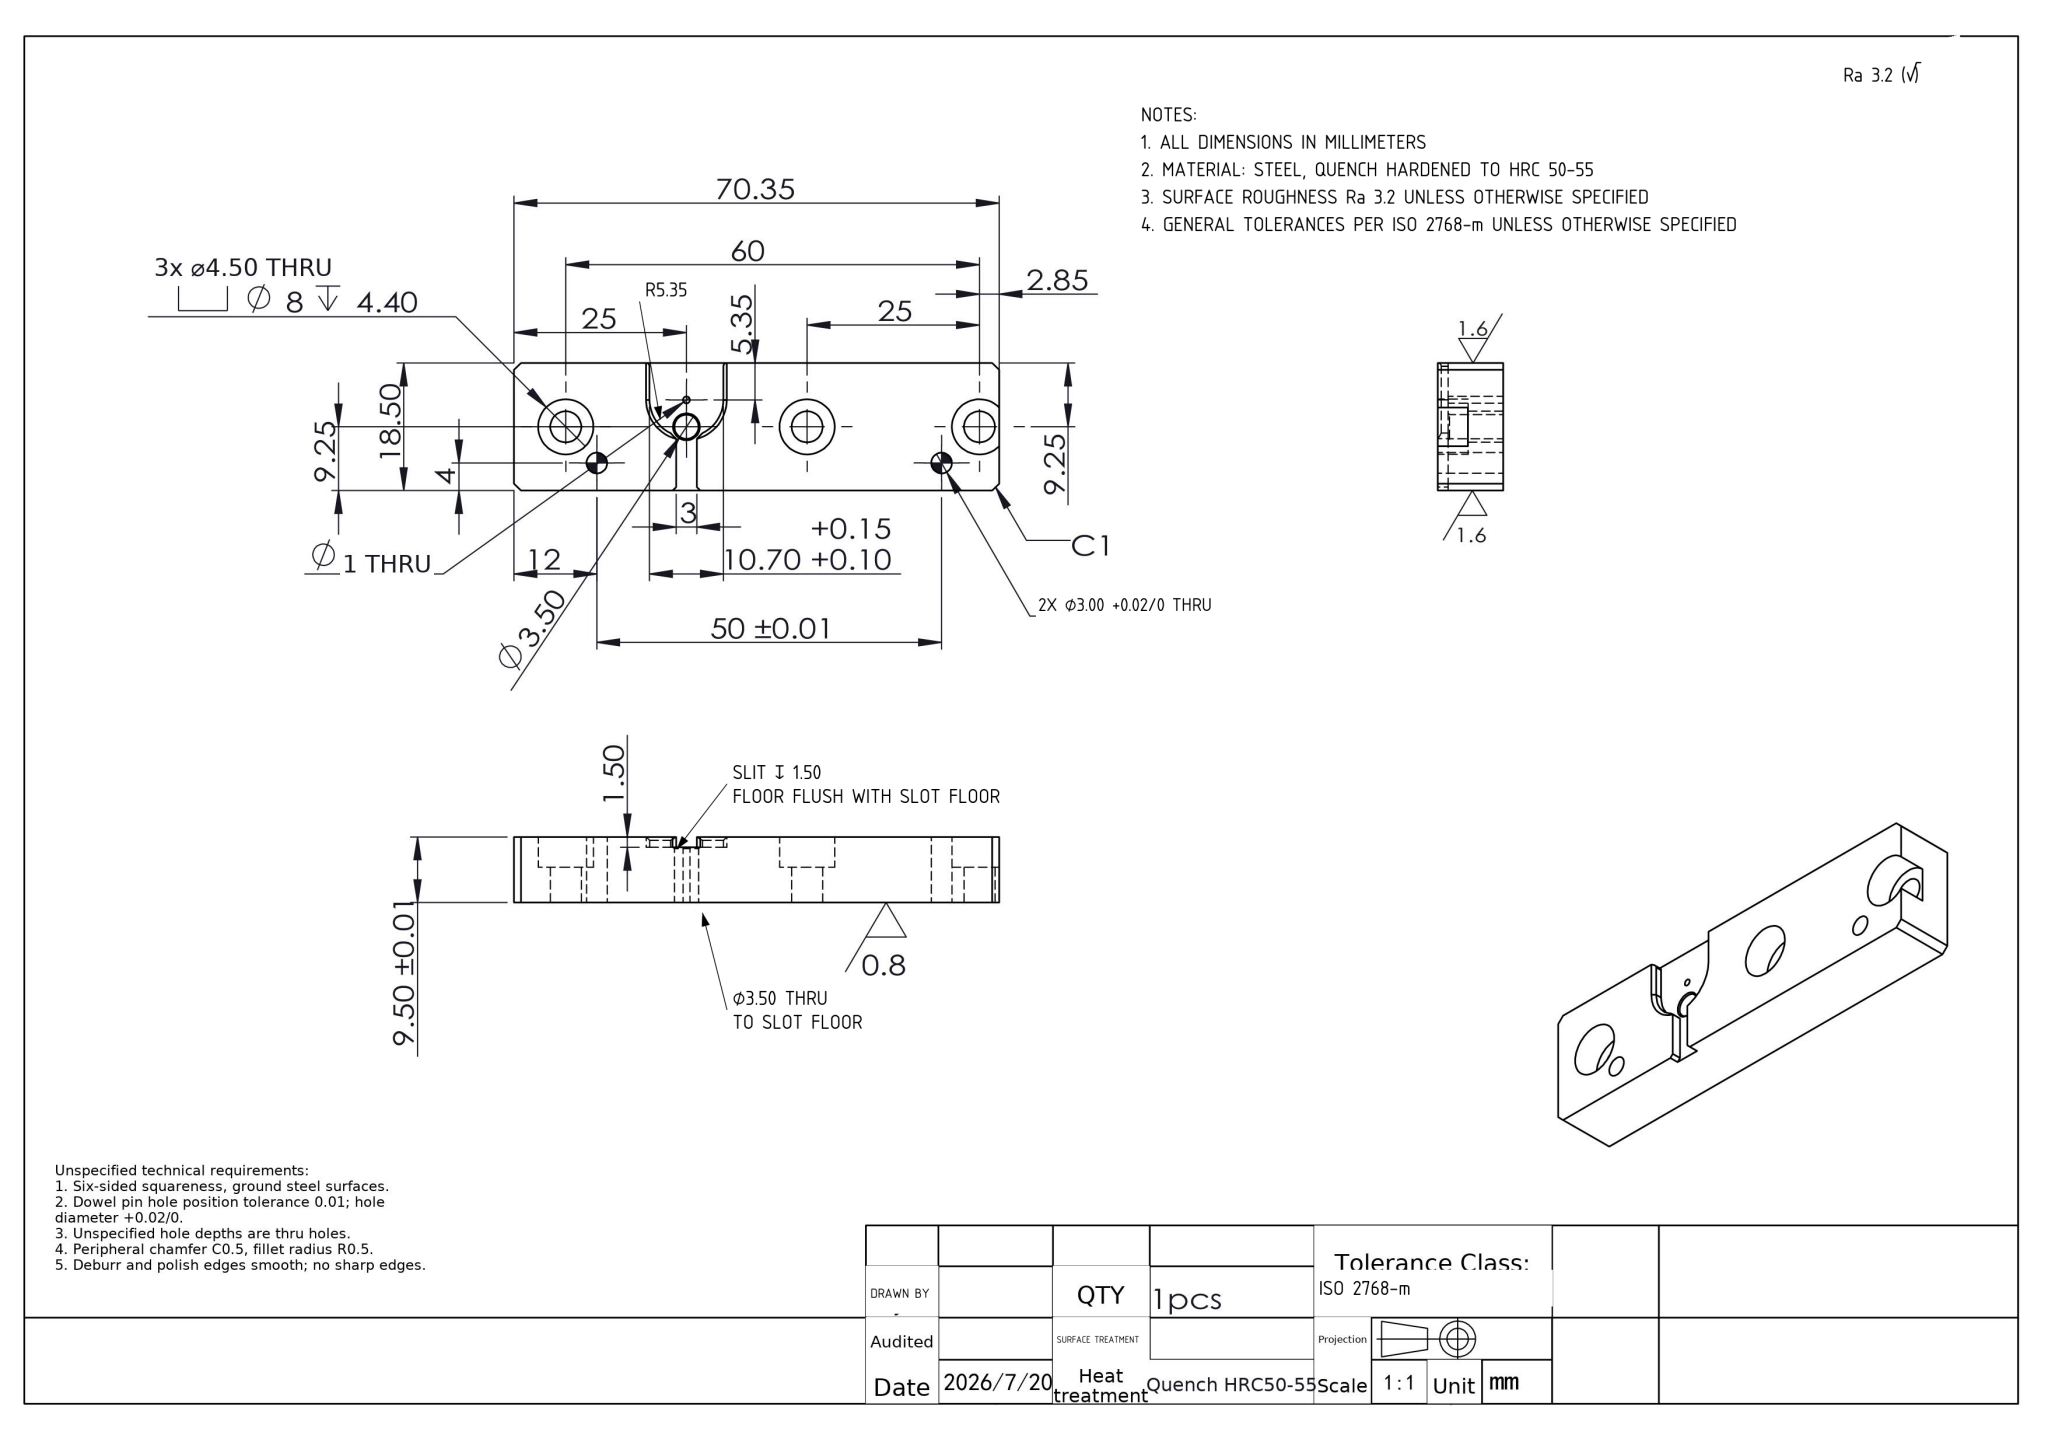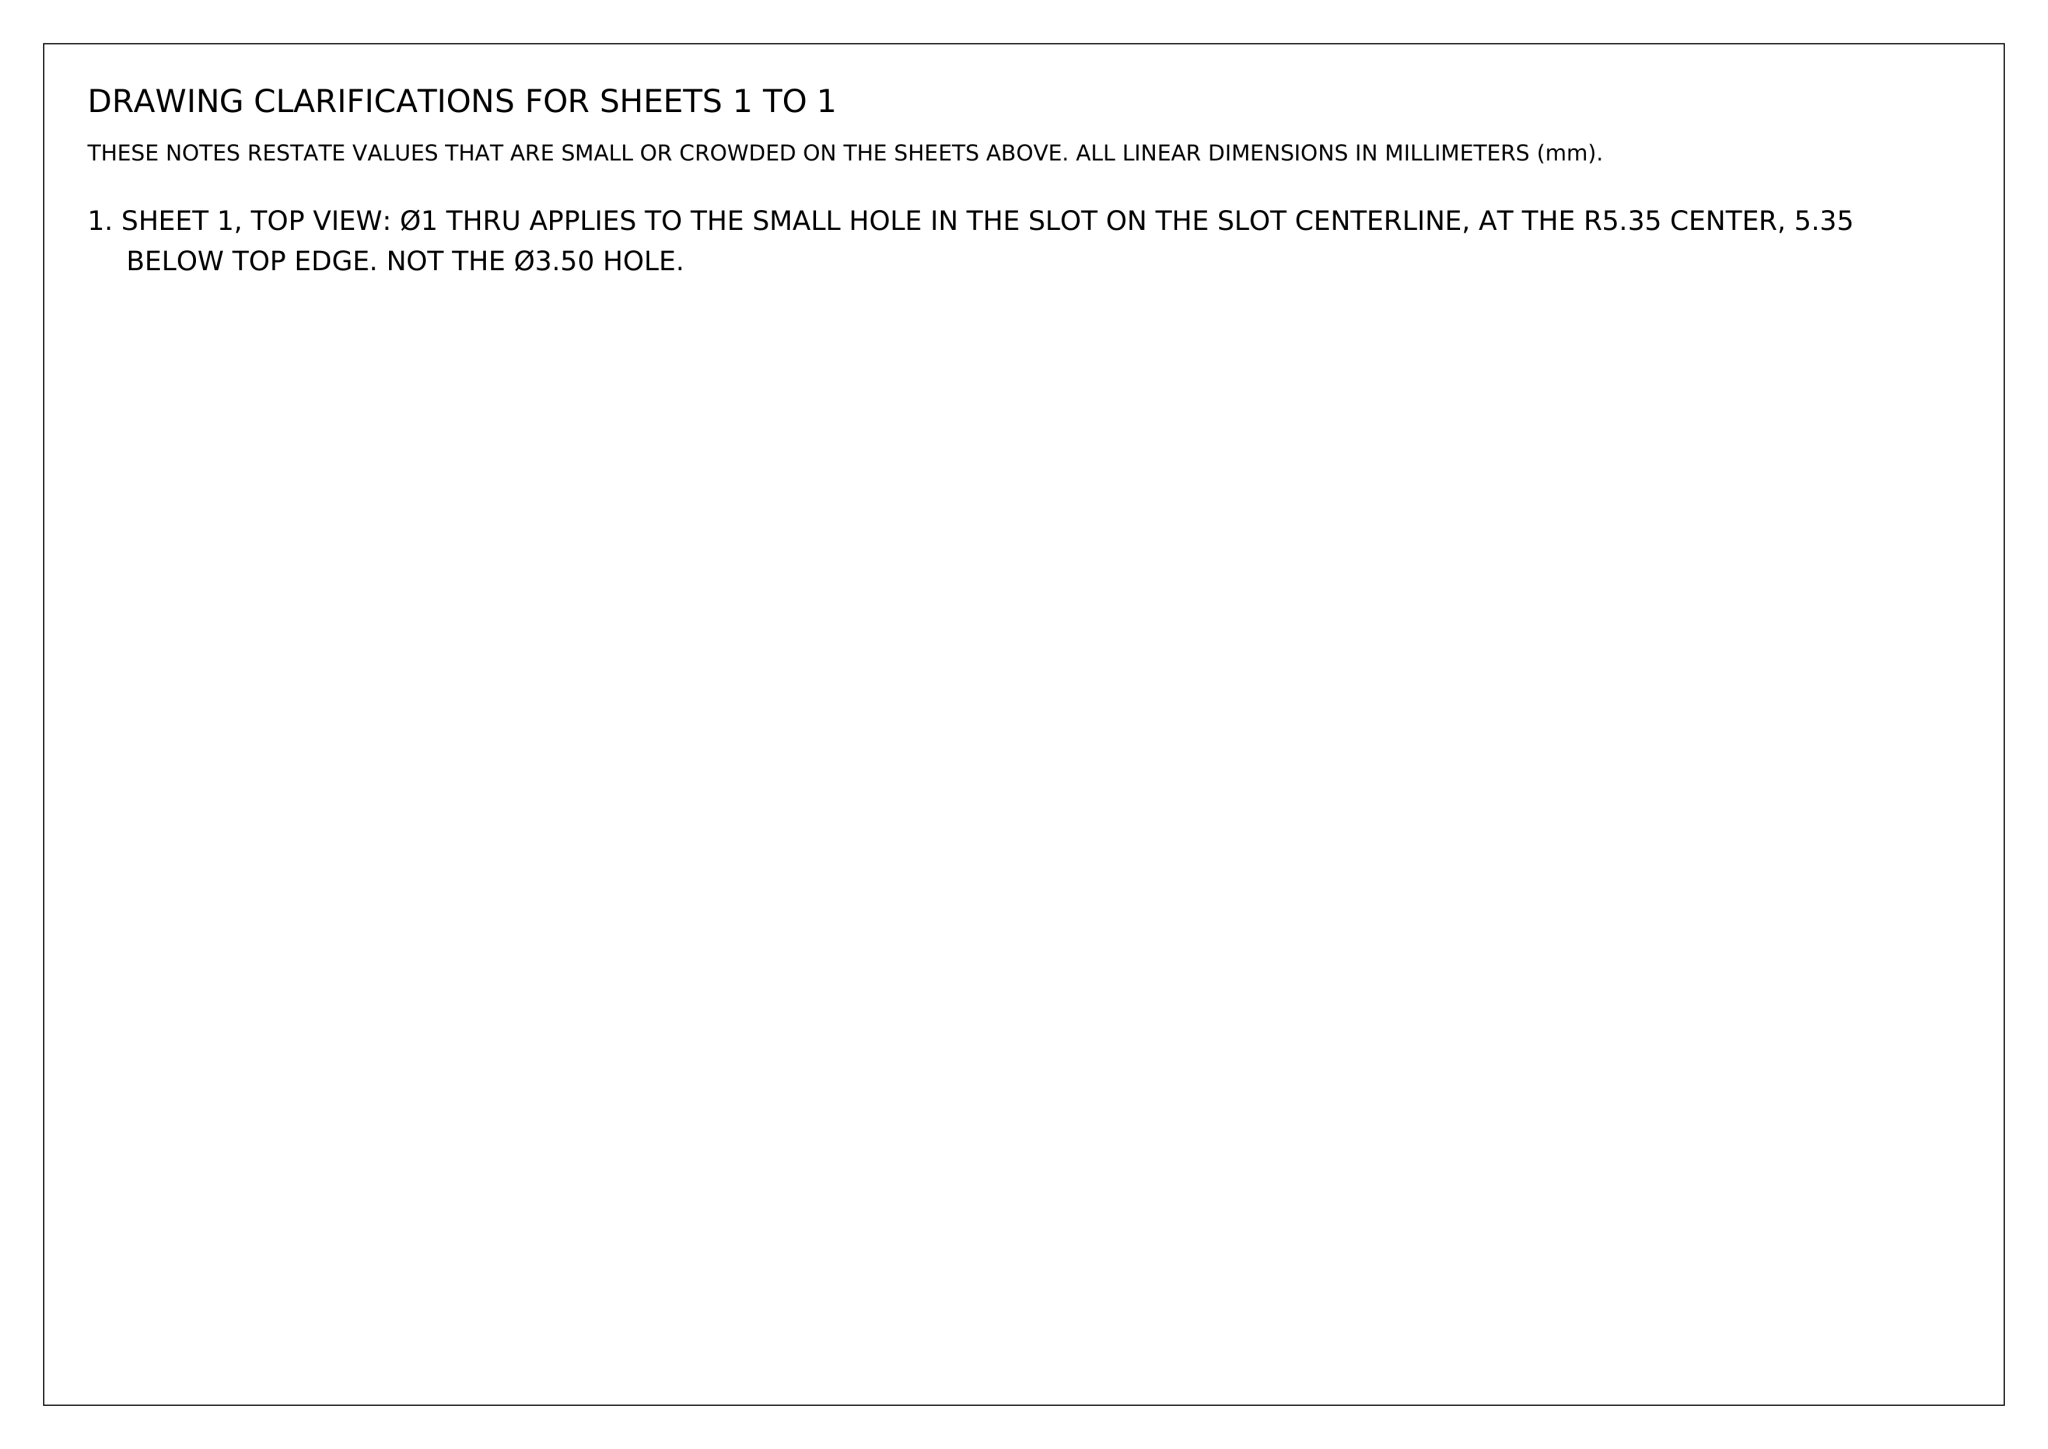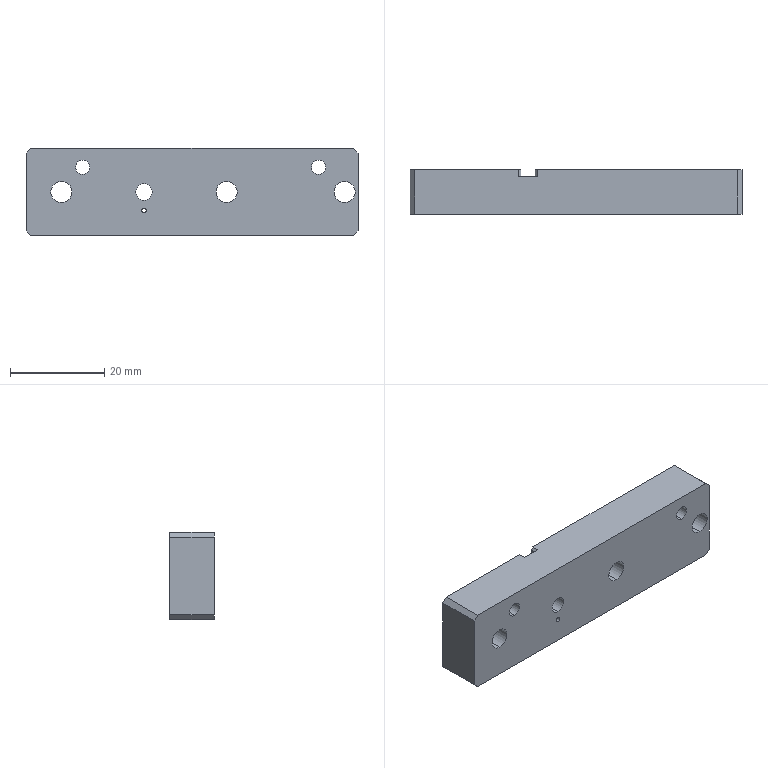Part | NX | mm | 1 solid | 54 faces | box 70.35 x 9.5 x 18.5 mm | volume 11047 mm3 | cylinder 25 | plane 25 | cone 4 | commonest cylinder face diameters 8 x7 4.5 x6 3 x4 1 x4 3.5 x2 10.7 x2